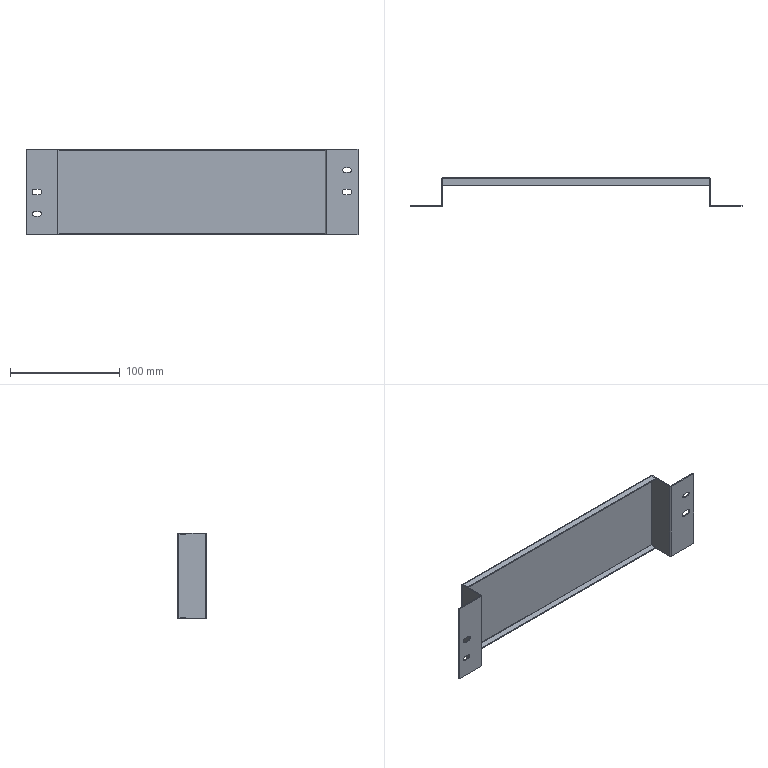Component | SolidWorks | Lampshade-1_Lampshade2-1 | 1 solid | 78 faces | volume 30106 mm3 | plane 54 | cylinder 24 | commonest cylinder face diameters 4 x6 5 x6 2.2 x6 0.2 x6